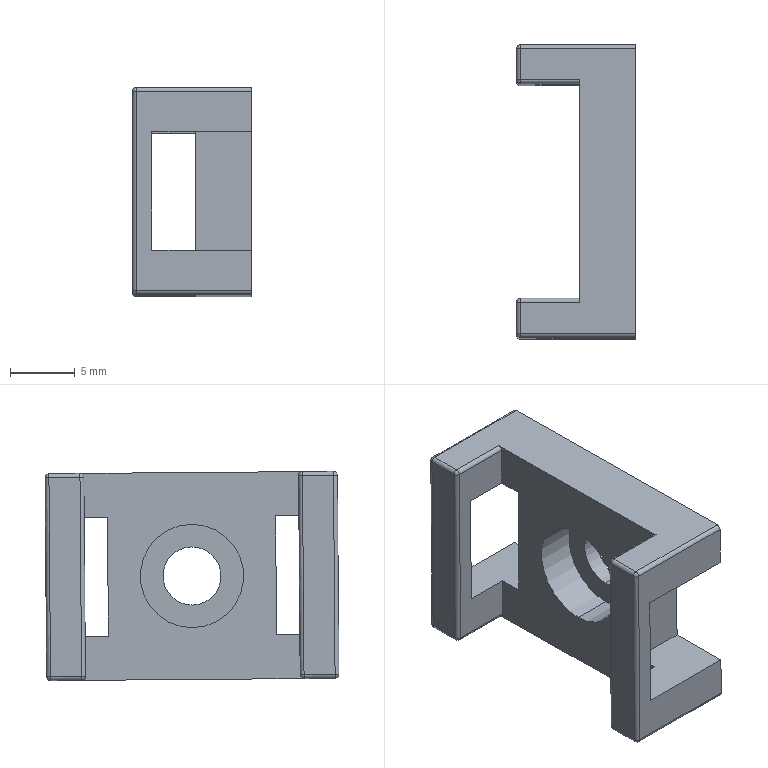Component | SolidWorks | WireClip~M4-02~-1111-15 | 1 solid | 47 faces | box 9.2 x 22.72 x 16.17 mm | volume 1284 mm3 | cylinder 20 | plane 19 | sphere 8 | commonest cylinder face diameters 0.6 x16 8 x2 4.5 x2 | material PEEK
build123d program:
from build123d import *

# Parameters (mm, degrees)
SKETCH1_W                                       = 22.6
SKETCH1_H                                       = 16
BOSS_EXTRUDE1_DEPTH                             = 9.2
SKETCH2_W                                       = 16.6
SKETCH2_H                                       = 4.9
CUT_EXTRUDE1_DEPTH                              = 30.179
SKETCH3_W                                       = 4.8
SKETCH3_H                                       = 9.2
CUT_EXTRUDE2_DEPTH                              = 7.7
M4_HEX_SOCKET_HEAD_CAP_SCREW_CBORE1_D           = 4.5
M4_HEX_SOCKET_HEAD_CAP_SCREW_CBORE1_CBORE_D     = 8
M4_HEX_SOCKET_HEAD_CAP_SCREW_CBORE1_CBORE_DEPTH = 3
FILLET1_R                                       = 0.3


with BuildPart() as part:
    # Sketch1 → Boss-Extrude1 (new body)
    with BuildSketch(Plane(origin=(0, 0, 0), x_dir=(1, 0, 0), z_dir=(0, 1, 0))):
        with Locations((11.3, 8)):
            Rectangle(SKETCH1_W, SKETCH1_H)
    extrude(amount=BOSS_EXTRUDE1_DEPTH)

    # Sketch2 → Cut-Extrude1 (cut, through all)
    with BuildSketch(Plane.XY):
        with Locations((11.3, 6.75)):
            Rectangle(SKETCH2_W, SKETCH2_H)
    extrude(amount=-CUT_EXTRUDE1_DEPTH, mode=Mode.SUBTRACT)

    # Sketch3 → Cut-Extrude2 (cut)
    with BuildSketch(Plane.XZ):
        with Locations((2.4, -8)):
            Rectangle(SKETCH3_W, SKETCH3_H)
        with Locations((20.2, -8)):
            Rectangle(SKETCH3_W, SKETCH3_H)
    extrude(amount=-CUT_EXTRUDE2_DEPTH, mode=Mode.SUBTRACT)

    # M4 Hex Socket Head Cap Screw CBORE1 (through all)
    with Locations(Plane(origin=(0, 4.3, 0), x_dir=(1, 0, 0), z_dir=(0, 1, 0))):
        with Locations((11.3, 8)):
            CounterBoreHole(M4_HEX_SOCKET_HEAD_CAP_SCREW_CBORE1_D / 2, M4_HEX_SOCKET_HEAD_CAP_SCREW_CBORE1_CBORE_D / 2, M4_HEX_SOCKET_HEAD_CAP_SCREW_CBORE1_CBORE_DEPTH)

    # Fillet1
    fillet1_edges = [part.edges().sort_by_distance(p)[0] for p in [
        (22.6, 9.2, -8),
        (21.1, 9.2, -16),
        (21.1, 9.2, 0),
        (1.5, 9.2, -16),
        (3, 6.75, -16),
        (3, 9.2, -8),
        (19.6, 6.75, -16),
        (19.6, 9.2, -8),
        (3, 6.75, 0),
        (19.6, 6.75, 0),
        (0, 9.2, -8),
        (1.5, 9.2, 0),
        (0, 4.6, -16),
        (22.6, 4.6, -16),
        (22.6, 4.6, 0),
        (0, 4.6, 0),
    ]]
    fillet(fillet1_edges, radius=FILLET1_R)


solid = part.part

# Placed as in the assembly
solid = solid.moved(Location((-165.072, 519.461, 1484.966), (179.545, 0, 90)))